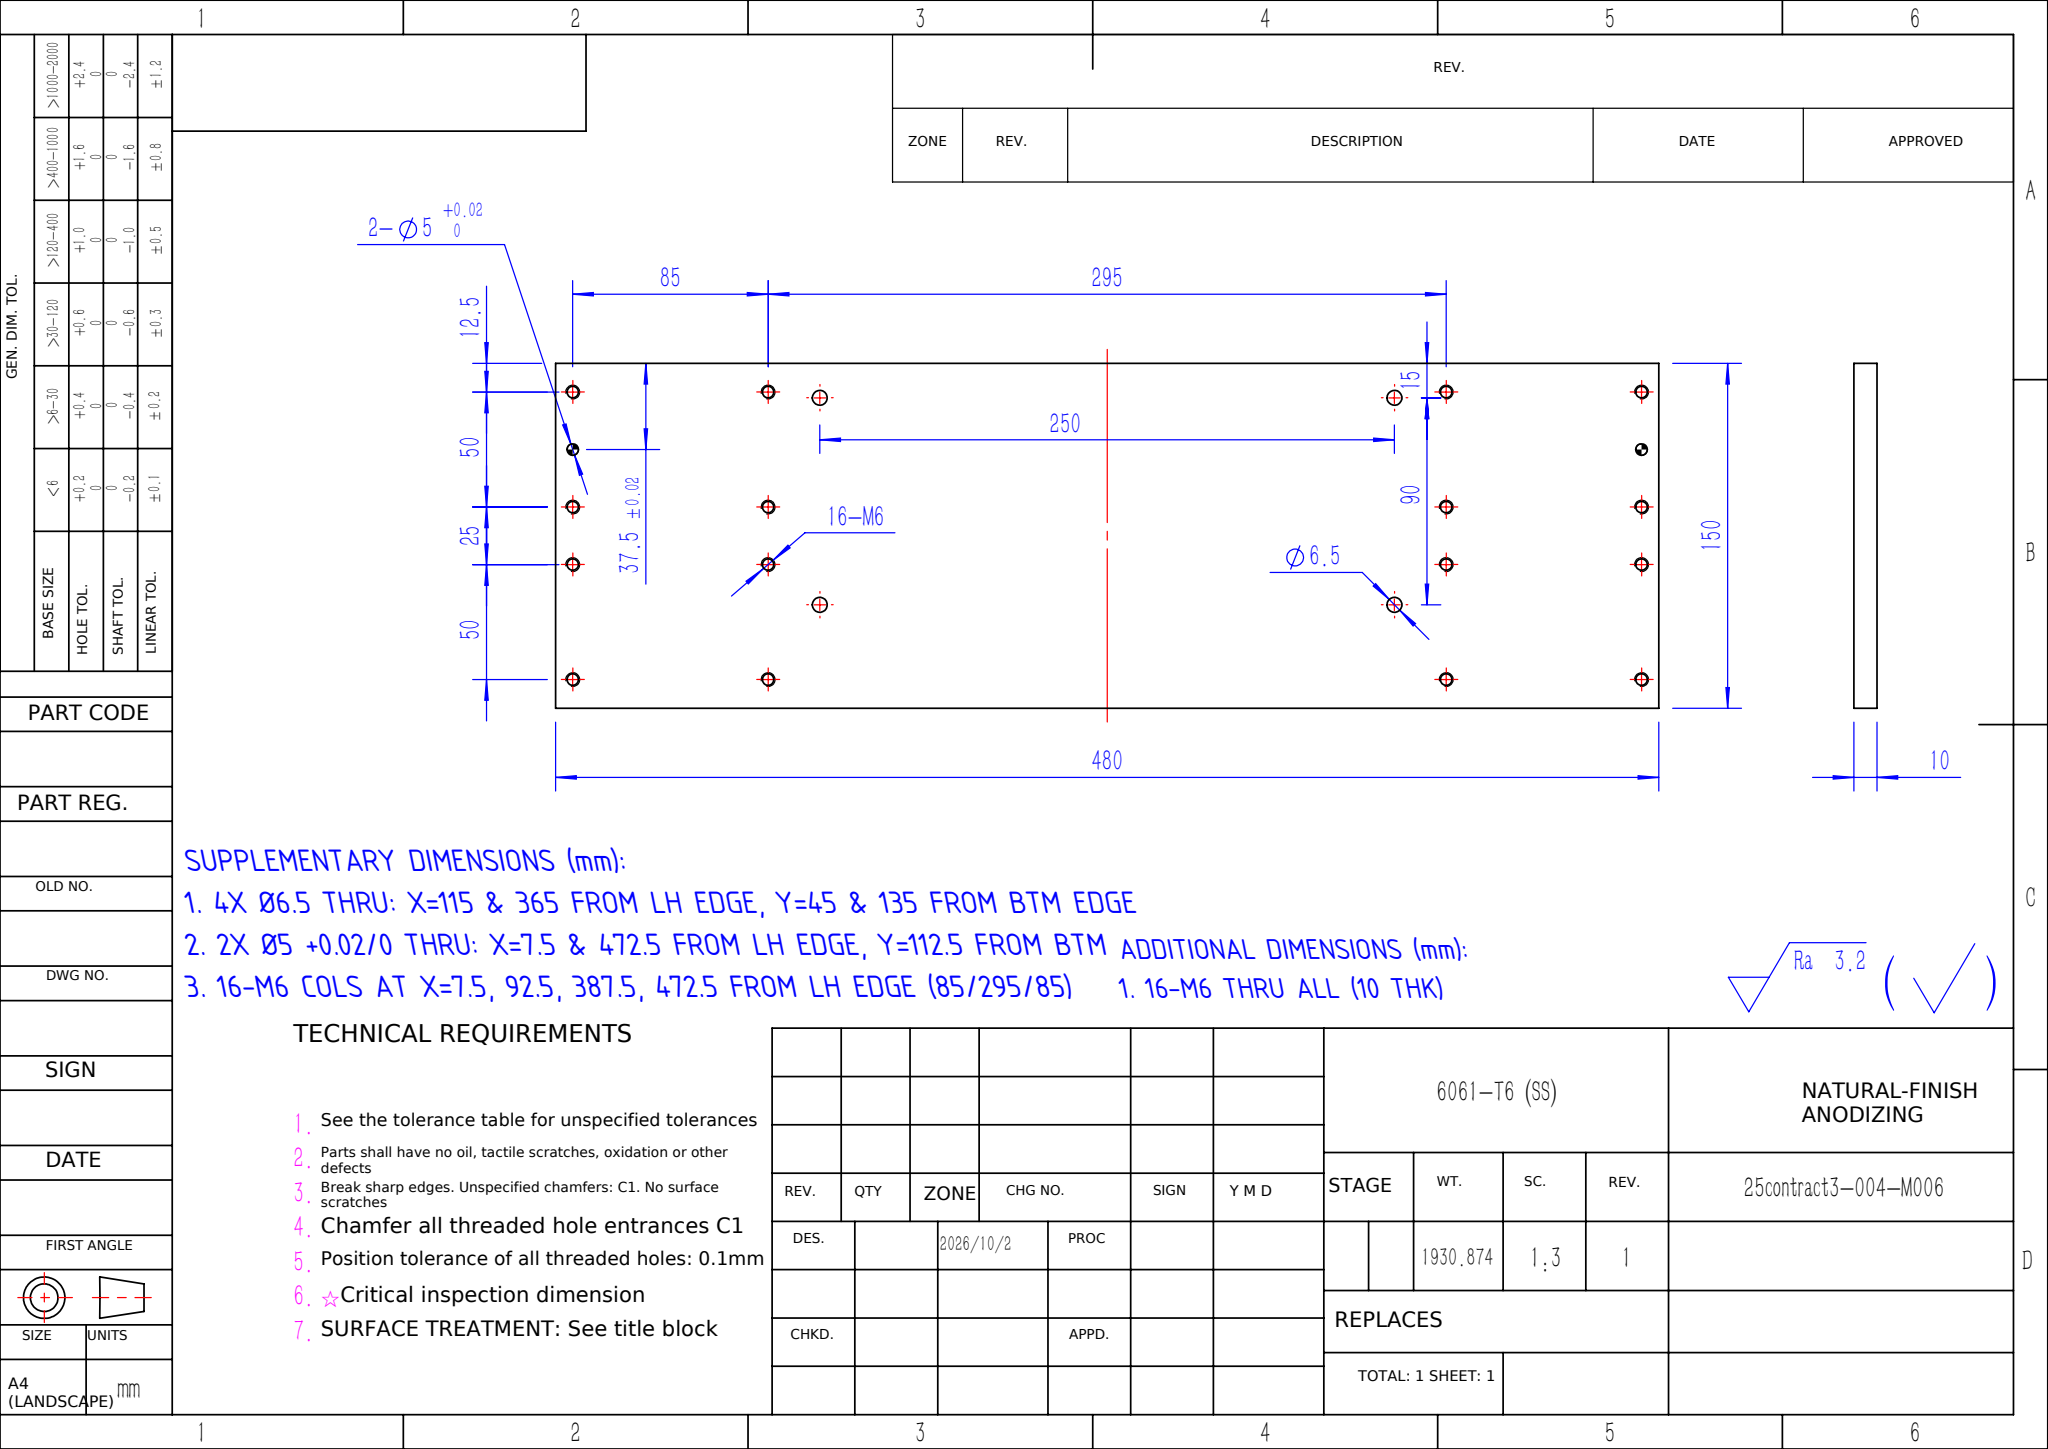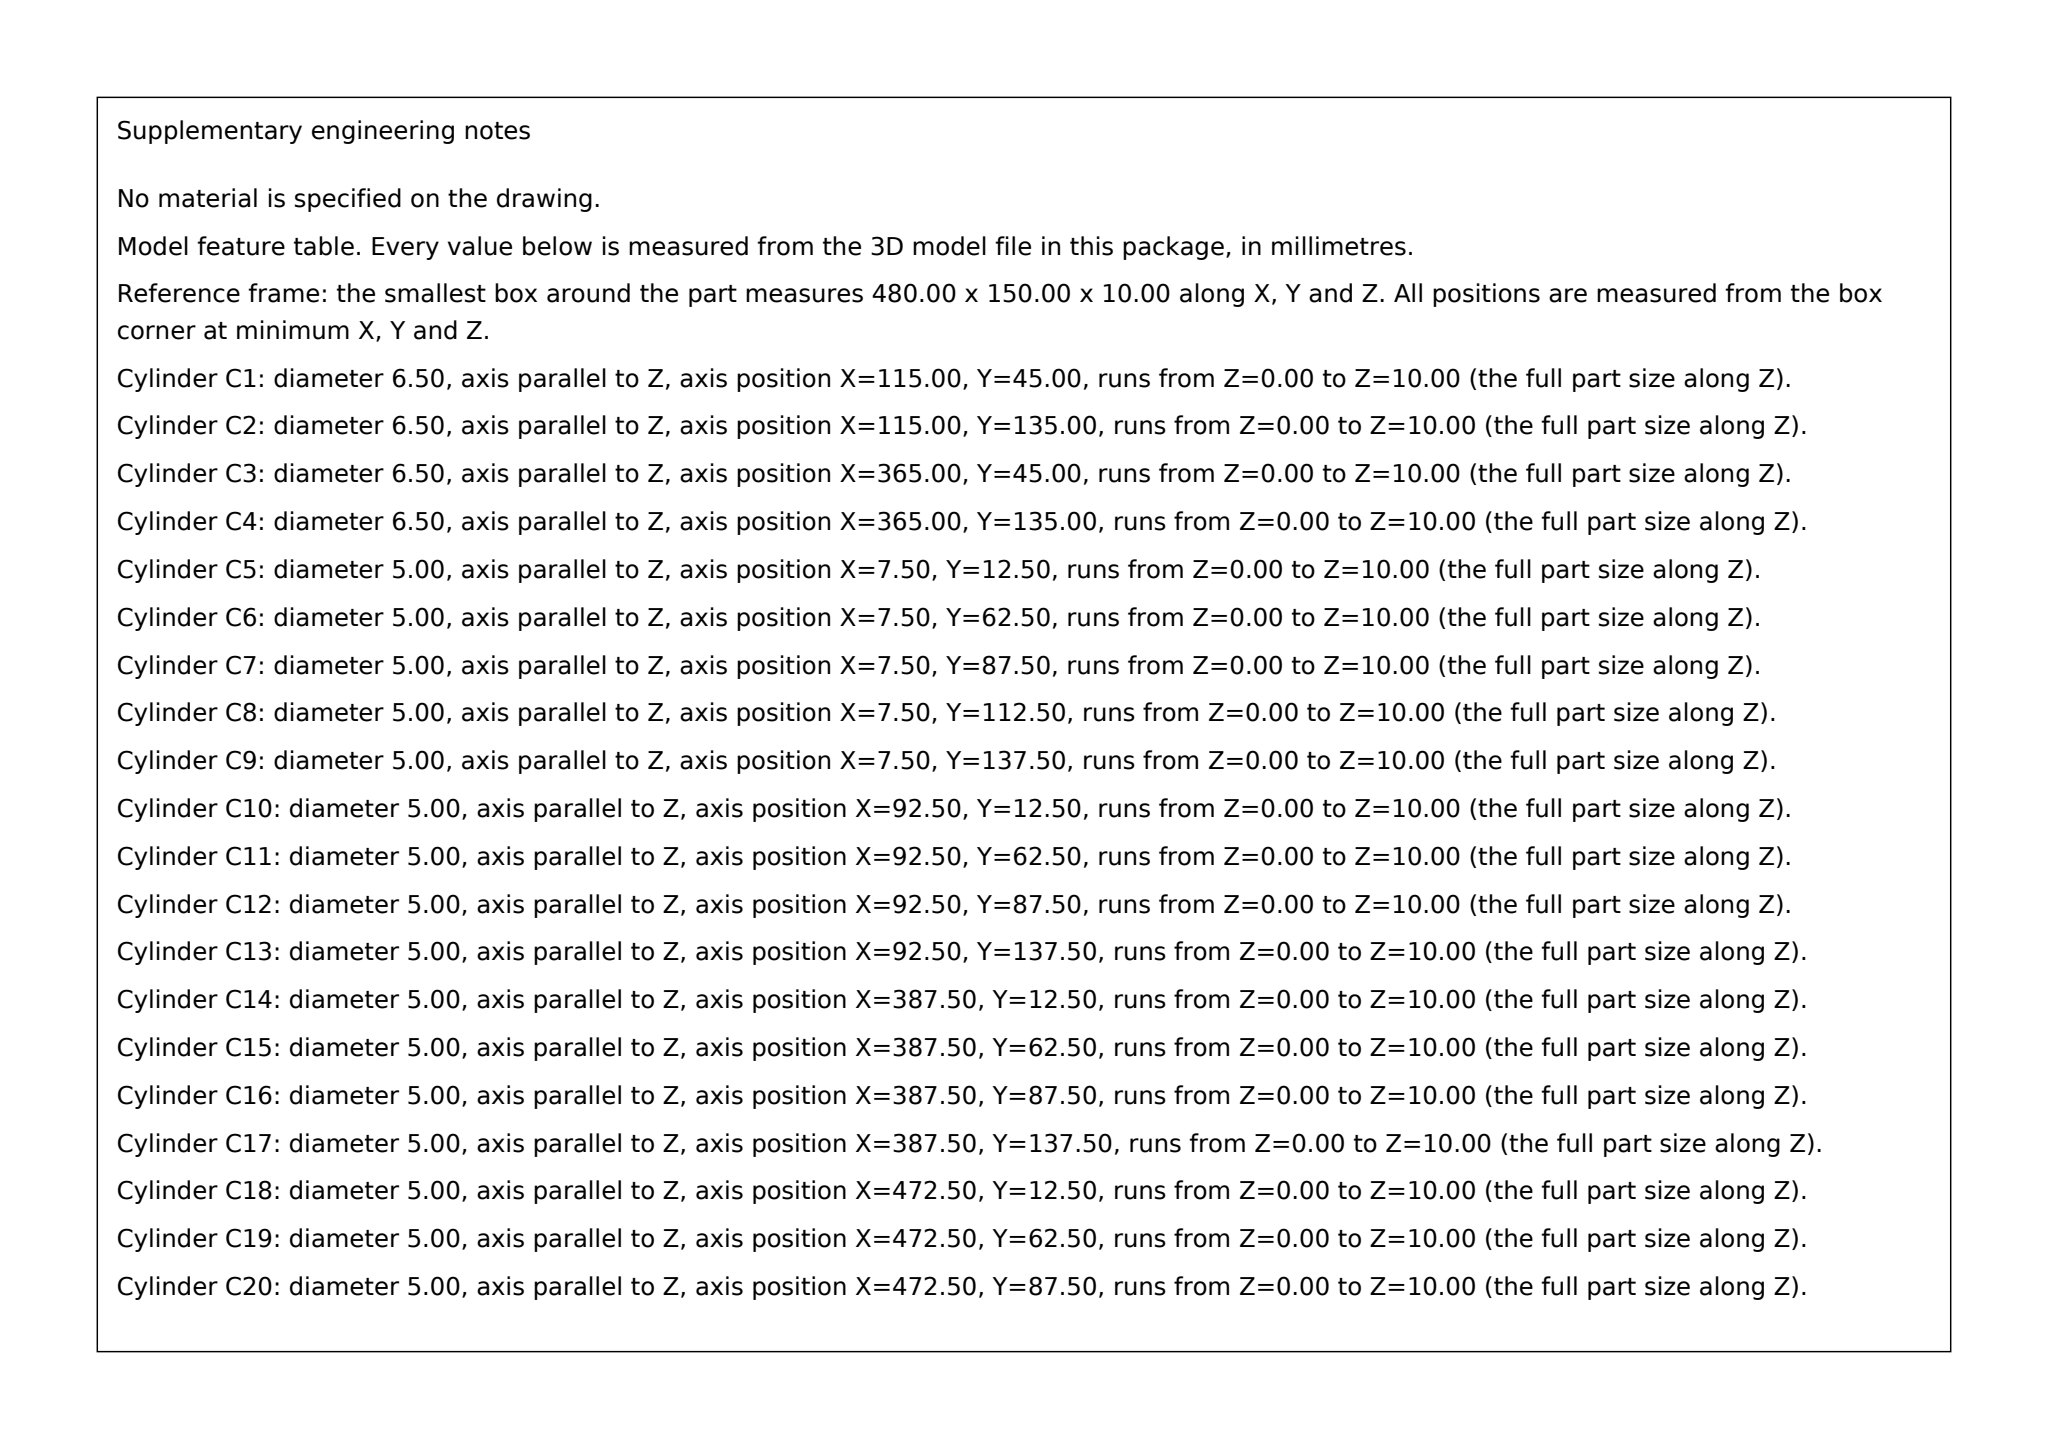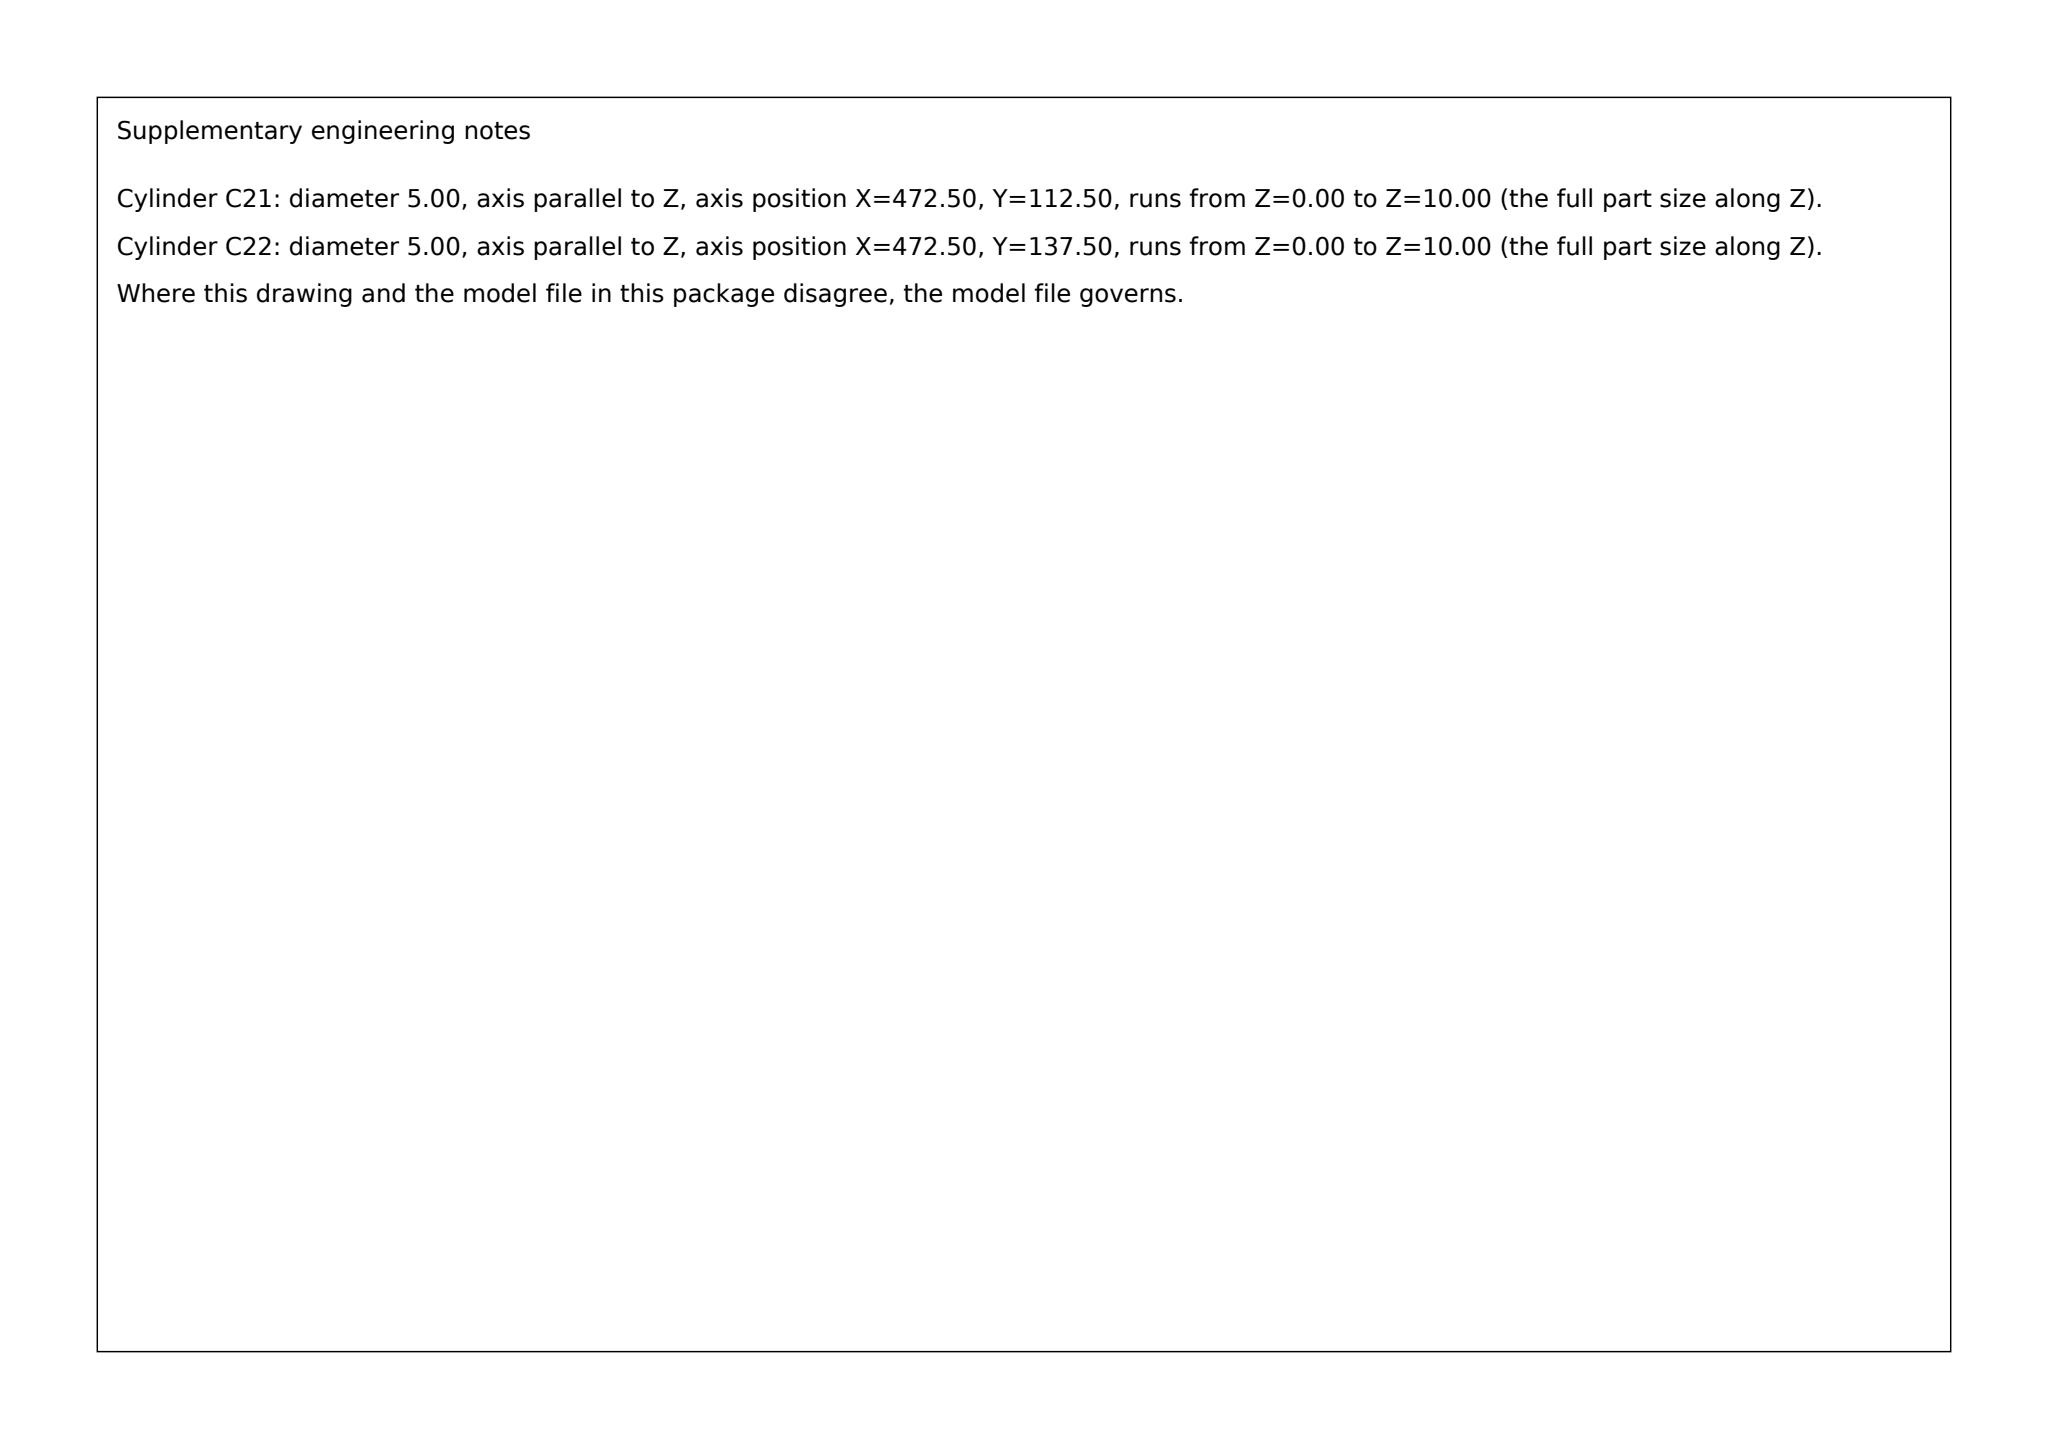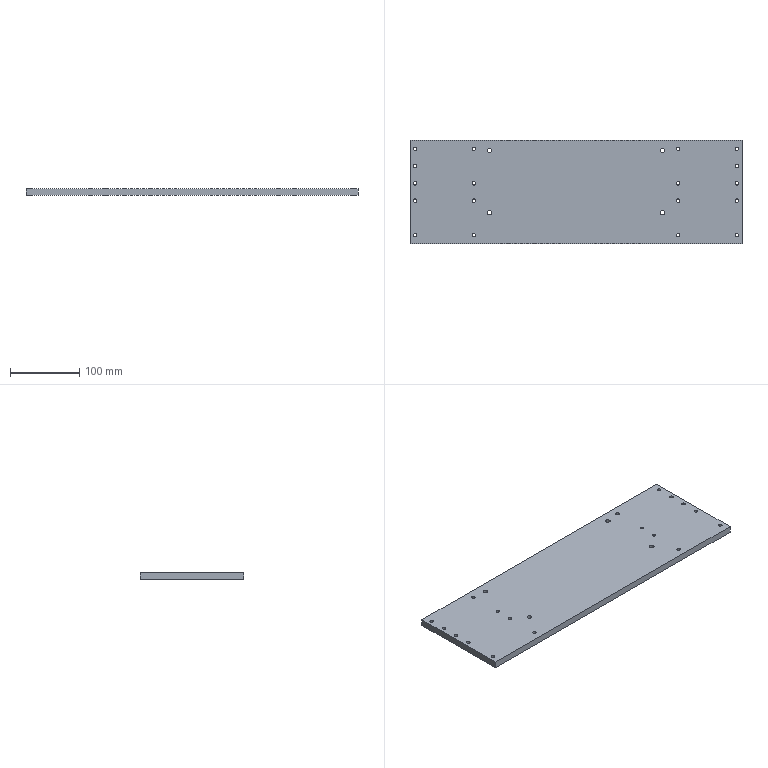Part | SolidWorks | mm | 1 solid | 50 faces | box 480 x 150 x 10 mm | volume 715138 mm3 | cylinder 44 | plane 6 | commonest cylinder face diameters 5 x36 6.5 x8
build123d program:
from build123d import *

# Parameters (mm, degrees)
SKETCH1_W                  = 480
SKETCH1_H                  = 150
BOSS_EXTRUDE1_DEPTH        = 10
M6_TAPPED_HOLE1_D          = 5
SIZE_MM_DOWEL_PIN_HOLE_1_D = 5
SIZE_MM_DOWEL_PIN_HOLE_2_D = 5
F_6_5_6_5_DIAMETER_HOLE1_D = 6.5
F_6_5_6_5_DIAMETER_HOLE2_D = 6.5


with BuildPart() as part:
    # Sketch1 → Boss-Extrude1 (new body)
    with BuildSketch(Plane.XY):
        Rectangle(SKETCH1_W, SKETCH1_H)
    extrude(amount=BOSS_EXTRUDE1_DEPTH)

    # M6 Tapped Hole1 (through all)
    with Locations(Plane.XY.offset(10)):
        with Locations((-147.5, 12.5), (-147.5, 62.5), (-232.5, 12.5), (-232.5, 62.5), (-147.5, -62.5), (-147.5, -12.5), (-232.5, -62.5), (-232.5, -12.5), (232.5, 12.5), (232.5, 62.5), (147.5, 12.5), (147.5, 62.5), (232.5, -62.5), (232.5, -12.5), (147.5, -62.5), (147.5, -12.5)):
            Hole(M6_TAPPED_HOLE1_D / 2)

    # Size mm Dowel Pin Hole 1 (through all)
    with Locations(Plane.XY.offset(10)):
        with Locations((-232.5, 37.5)):
            Hole(SIZE_MM_DOWEL_PIN_HOLE_1_D / 2)

    # Size mm Dowel Pin Hole 2 (through all)
    with Locations(Plane.XY.offset(10)):
        with Locations((232.5, 37.5)):
            Hole(SIZE_MM_DOWEL_PIN_HOLE_2_D / 2)

    # 6.5 _6.5_ Diameter Hole1 (through all)
    with Locations(Plane.XY.offset(10)):
        with Locations((-125, -30), (-125, 60)):
            Hole(F_6_5_6_5_DIAMETER_HOLE1_D / 2)

    # 6.5 _6.5_ Diameter Hole2 (through all)
    with Locations(Plane.XY.offset(10)):
        with Locations((125, -30), (125, 60)):
            Hole(F_6_5_6_5_DIAMETER_HOLE2_D / 2)


solid = part.part